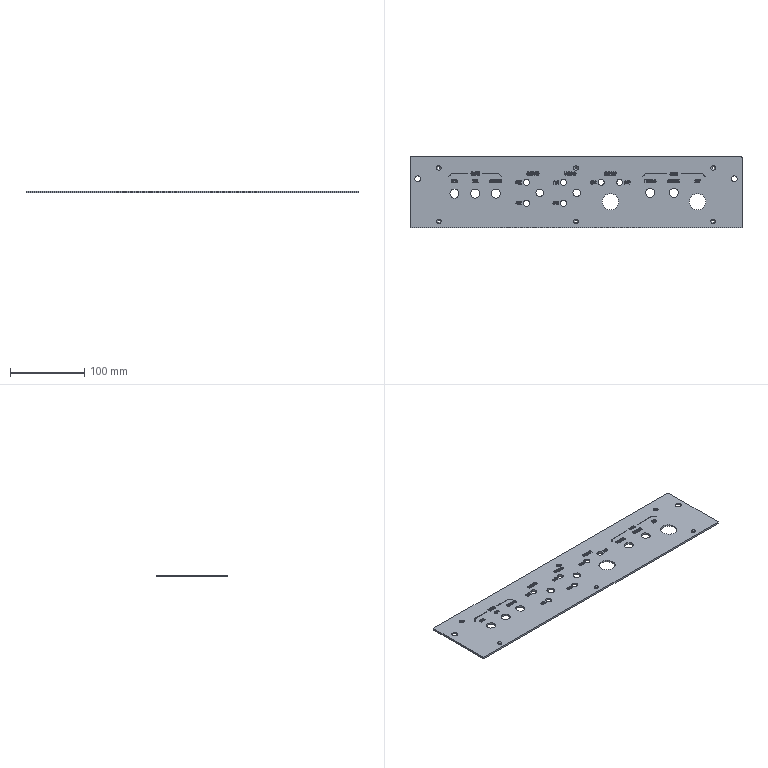CAM job | Mastercam | mm | 7 operations | part box 448 x 95.85 x 2.5
1. Contour (Ramp) | 9 - 10 平铣刀
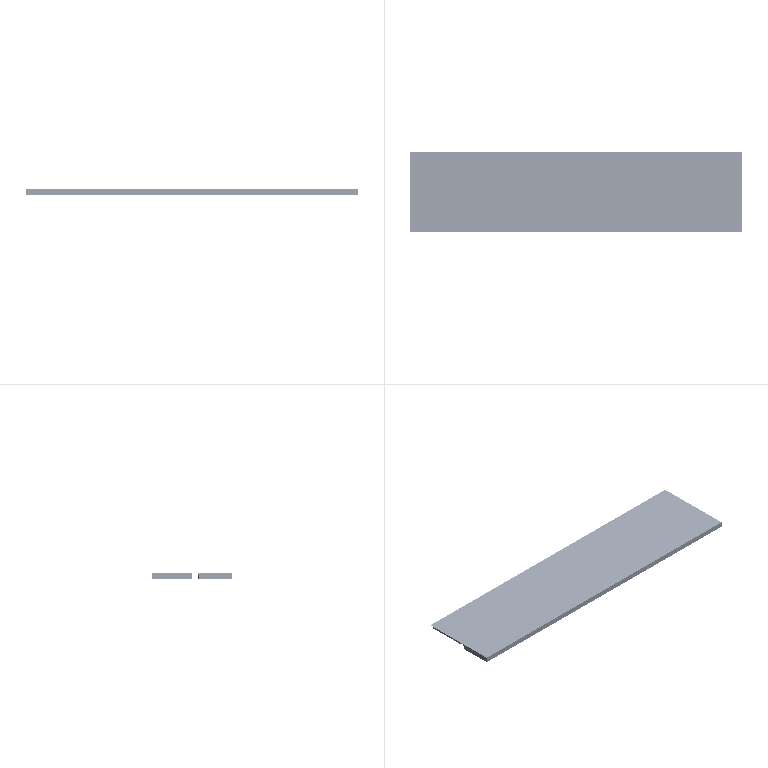2. Contour (2D) | 10 - 10 平铣刀
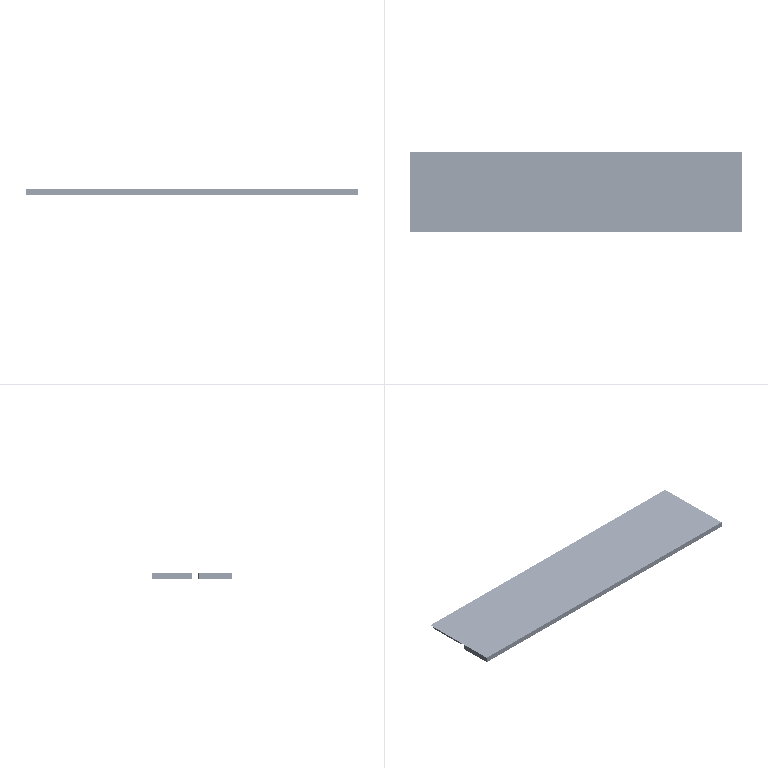3. Surface Finish Flowline | 4 - 4 平铣刀
4. Contour (Ramp) | 4 - 4 平铣刀
5. Contour (2D) | 3 - 3 平铣刀
6. Contour (2D chamfer) | 5 - 4 倒角刀
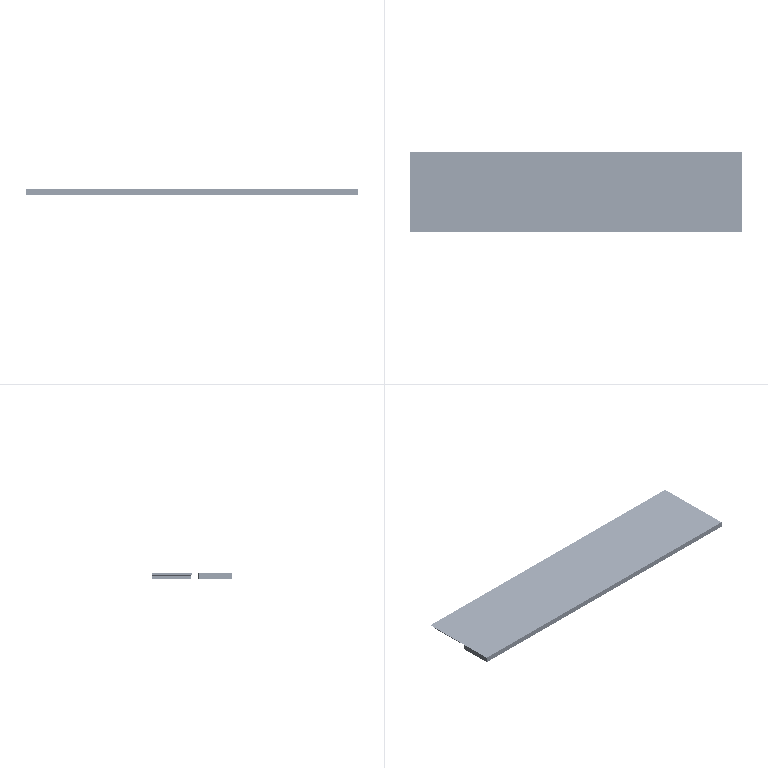7. Drill/Counterbore | 5 - 4 倒角刀